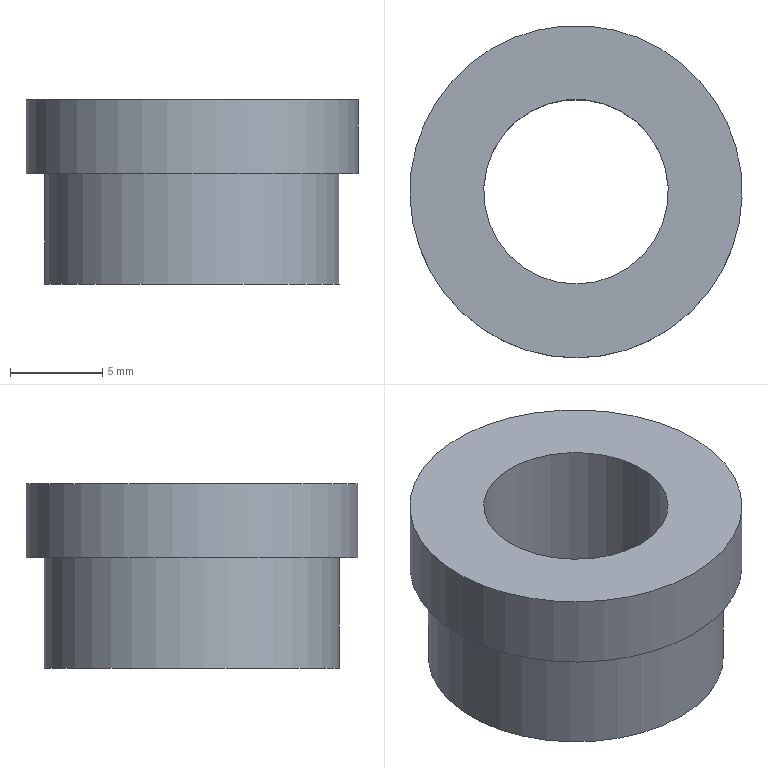Component | NX | GLAND | 1 solid | 6 faces | box 18 x 18 x 10 mm | volume 1341 mm3 | cylinder 3 | plane 2 | cone 1 | commonest cylinder face diameters 16 x1 10 x1 18 x1
STEP:
#1=CARTESIAN_POINT('',(0.,0.,0.));
#2=DIRECTION('',(0.,0.,1.));
#3=DIRECTION('',(1.,0.,0.));
#4=AXIS2_PLACEMENT_3D('',#1,#2,#3);
#5=CARTESIAN_POINT('',(10.284,-2.216,132.));
#6=VERTEX_POINT('',#5);
#7=CARTESIAN_POINT('',(10.284,5.784,132.));
#8=DIRECTION('',(0.,0.,1.));
#9=DIRECTION('',(0.,-1.,0.));
#10=AXIS2_PLACEMENT_3D('',#7,#8,#9);
#11=CIRCLE('',#10,8.);
#12=CARTESIAN_POINT('',(10.284,5.784,132.));
#13=DIRECTION('',(0.,0.,1.));
#14=DIRECTION('',(0.,-1.,0.));
#15=AXIS2_PLACEMENT_3D('',#12,#13,#14);
#16=CYLINDRICAL_SURFACE('',#15,8.);
#17=CARTESIAN_POINT('',(0.,0.));
#18=DIRECTION('',(1.,0.));
#19=VECTOR('',#18,1.);
#20=LINE('',#17,#19);
#21=(GEOMETRIC_REPRESENTATION_CONTEXT(2)PARAMETRIC_REPRESENTATION_CONTEXT()REPRESENTATION_CONTEXT('',''));
#22=DEFINITIONAL_REPRESENTATION('',(#20),#21);
#23=PCURVE('',#16,#22);
#24=CARTESIAN_POINT('',(10.284,5.784,132.));
#25=DIRECTION('',(0.,-0.,-1.));
#26=DIRECTION('',(0.,1.,-0.));
#27=AXIS2_PLACEMENT_3D('',#24,#25,#26);
#28=CONICAL_SURFACE('',#27,8.,1.047);
#29=CARTESIAN_POINT('',(9.425,0.));
#30=DIRECTION('',(-1.,0.));
#31=VECTOR('',#30,1.);
#32=LINE('',#29,#31);
#33=(GEOMETRIC_REPRESENTATION_CONTEXT(2)PARAMETRIC_REPRESENTATION_CONTEXT()REPRESENTATION_CONTEXT('',''));
#34=DEFINITIONAL_REPRESENTATION('',(#32),#33);
#35=PCURVE('',#28,#34);
#36=SURFACE_CURVE('',#11,(#23,#35),.PCURVE_S1.);
#37=EDGE_CURVE('',#6,#6,#36,.T.);
#38=ORIENTED_EDGE('',*,*,#37,.T.);
#39=CARTESIAN_POINT('',(10.284,-2.216,138.));
#40=VERTEX_POINT('',#39);
#41=CARTESIAN_POINT('',(10.284,-2.216,132.));
#42=CARTESIAN_POINT('',(10.284,-2.216,138.));
#43=B_SPLINE_CURVE_WITH_KNOTS('',1,(#41,#42),.UNSPECIFIED.,.F.,.F.,(2,2),(0.,6.),.PIECEWISE_BEZIER_KNOTS.);
#44=CARTESIAN_POINT('',(6.283,0.));
#45=DIRECTION('',(0.,1.));
#46=VECTOR('',#45,1.);
#47=LINE('',#44,#46);
#48=(GEOMETRIC_REPRESENTATION_CONTEXT(2)PARAMETRIC_REPRESENTATION_CONTEXT()REPRESENTATION_CONTEXT('',''));
#49=DEFINITIONAL_REPRESENTATION('',(#47),#48);
#50=PCURVE('',#16,#49);
#51=CARTESIAN_POINT('',(0.,0.));
#52=DIRECTION('',(0.,1.));
#53=VECTOR('',#52,1.);
#54=LINE('',#51,#53);
#55=(GEOMETRIC_REPRESENTATION_CONTEXT(2)PARAMETRIC_REPRESENTATION_CONTEXT()REPRESENTATION_CONTEXT('',''));
#56=DEFINITIONAL_REPRESENTATION('',(#54),#55);
#57=PCURVE('',#16,#56);
#58=SEAM_CURVE('',#43,(#50,#57),.PCURVE_S1.);
#59=EDGE_CURVE('',#6,#40,#58,.T.);
#60=ORIENTED_EDGE('',*,*,#59,.T.);
#61=CARTESIAN_POINT('',(10.284,5.784,138.));
#62=DIRECTION('',(0.,0.,1.));
#63=DIRECTION('',(0.,-1.,0.));
#64=AXIS2_PLACEMENT_3D('',#61,#62,#63);
#65=CIRCLE('',#64,8.);
#66=CARTESIAN_POINT('',(0.,6.));
#67=DIRECTION('',(1.,0.));
#68=VECTOR('',#67,1.);
#69=LINE('',#66,#68);
#70=(GEOMETRIC_REPRESENTATION_CONTEXT(2)PARAMETRIC_REPRESENTATION_CONTEXT()REPRESENTATION_CONTEXT('',''));
#71=DEFINITIONAL_REPRESENTATION('',(#69),#70);
#72=PCURVE('',#16,#71);
#73=CARTESIAN_POINT('',(10.284,14.784,138.));
#74=DIRECTION('',(0.,-0.,-1.));
#75=DIRECTION('',(0.,1.,-0.));
#76=AXIS2_PLACEMENT_3D('',#73,#74,#75);
#77=PLANE('',#76);
#78=CARTESIAN_POINT('',(-17.,0.));
#79=CARTESIAN_POINT('',(-17.,13.856));
#80=CARTESIAN_POINT('',(-5.,6.928));
#81=CARTESIAN_POINT('',(7.,0.));
#82=CARTESIAN_POINT('',(-5.,-6.928));
#83=CARTESIAN_POINT('',(-17.,-13.856));
#84=CARTESIAN_POINT('',(-17.,0.));
#85=(BOUNDED_CURVE()B_SPLINE_CURVE(2,(#78,#79,#80,#81,#82,#83,#84),.UNSPECIFIED.,.T.,.F.)B_SPLINE_CURVE_WITH_KNOTS((1,2,2,2,2,1),(-2.094,0.,2.094,4.189,6.283,8.378),.UNSPECIFIED.)CURVE()GEOMETRIC_REPRESENTATION_ITEM()RATIONAL_B_SPLINE_CURVE((1.,0.5,1.,0.5,1.,0.5,1.))REPRESENTATION_ITEM(''));
#86=(GEOMETRIC_REPRESENTATION_CONTEXT(2)PARAMETRIC_REPRESENTATION_CONTEXT()REPRESENTATION_CONTEXT('',''));
#87=DEFINITIONAL_REPRESENTATION('',(#85),#86);
#88=PCURVE('',#77,#87);
#89=SURFACE_CURVE('',#65,(#72,#88),.PCURVE_S1.);
#90=EDGE_CURVE('',#40,#40,#89,.T.);
#91=ORIENTED_EDGE('',*,*,#90,.F.);
#92=ORIENTED_EDGE('',*,*,#59,.F.);
#93=EDGE_LOOP('',(#38,#60,#91,#92));
#94=FACE_BOUND('',#93,.T.);
#95=ADVANCED_FACE('',(#94),#16,.T.);
#96=CARTESIAN_POINT('',(10.284,0.7843,133.732));
#97=VERTEX_POINT('',#96);
#98=CARTESIAN_POINT('',(10.284,5.784,133.732));
#99=DIRECTION('',(0.,0.,1.));
#100=DIRECTION('',(0.,-1.,0.));
#101=AXIS2_PLACEMENT_3D('',#98,#99,#100);
#102=CIRCLE('',#101,5.);
#103=CARTESIAN_POINT('',(9.425,-1.732));
#104=DIRECTION('',(-1.,0.));
#105=VECTOR('',#104,1.);
#106=LINE('',#103,#105);
#107=(GEOMETRIC_REPRESENTATION_CONTEXT(2)PARAMETRIC_REPRESENTATION_CONTEXT()REPRESENTATION_CONTEXT('',''));
#108=DEFINITIONAL_REPRESENTATION('',(#106),#107);
#109=PCURVE('',#28,#108);
#110=CARTESIAN_POINT('',(10.284,5.784,132.));
#111=DIRECTION('',(0.,0.,1.));
#112=DIRECTION('',(0.,-1.,0.));
#113=AXIS2_PLACEMENT_3D('',#110,#111,#112);
#114=CYLINDRICAL_SURFACE('',#113,5.);
#115=CARTESIAN_POINT('',(0.,1.732));
#116=DIRECTION('',(1.,0.));
#117=VECTOR('',#116,1.);
#118=LINE('',#115,#117);
#119=(GEOMETRIC_REPRESENTATION_CONTEXT(2)PARAMETRIC_REPRESENTATION_CONTEXT()REPRESENTATION_CONTEXT('',''));
#120=DEFINITIONAL_REPRESENTATION('',(#118),#119);
#121=PCURVE('',#114,#120);
#122=SURFACE_CURVE('',#102,(#109,#121),.PCURVE_S1.);
#123=EDGE_CURVE('',#97,#97,#122,.T.);
#124=ORIENTED_EDGE('',*,*,#123,.F.);
#125=CARTESIAN_POINT('',(10.284,0.7843,133.732));
#126=CARTESIAN_POINT('',(10.284,-2.216,132.));
#127=B_SPLINE_CURVE_WITH_KNOTS('',1,(#125,#126),.UNSPECIFIED.,.F.,.F.,(2,2),(-3.464,0.),.PIECEWISE_BEZIER_KNOTS.);
#128=CARTESIAN_POINT('',(9.425,0.));
#129=DIRECTION('',(0.,1.));
#130=VECTOR('',#129,1.);
#131=LINE('',#128,#130);
#132=(GEOMETRIC_REPRESENTATION_CONTEXT(2)PARAMETRIC_REPRESENTATION_CONTEXT()REPRESENTATION_CONTEXT('',''));
#133=DEFINITIONAL_REPRESENTATION('',(#131),#132);
#134=PCURVE('',#28,#133);
#135=CARTESIAN_POINT('',(3.142,0.));
#136=DIRECTION('',(0.,1.));
#137=VECTOR('',#136,1.);
#138=LINE('',#135,#137);
#139=(GEOMETRIC_REPRESENTATION_CONTEXT(2)PARAMETRIC_REPRESENTATION_CONTEXT()REPRESENTATION_CONTEXT('',''));
#140=DEFINITIONAL_REPRESENTATION('',(#138),#139);
#141=PCURVE('',#28,#140);
#142=SEAM_CURVE('',#127,(#134,#141),.PCURVE_S1.);
#143=EDGE_CURVE('',#97,#6,#142,.T.);
#144=ORIENTED_EDGE('',*,*,#143,.T.);
#145=ORIENTED_EDGE('',*,*,#37,.T.);
#146=ORIENTED_EDGE('',*,*,#143,.F.);
#147=EDGE_LOOP('',(#124,#144,#145,#146));
#148=FACE_BOUND('',#147,.F.);
#149=ADVANCED_FACE('',(#148),#28,.F.);
#150=CARTESIAN_POINT('',(10.284,0.7843,142.));
#151=VERTEX_POINT('',#150);
#152=CARTESIAN_POINT('',(10.284,5.784,142.));
#153=DIRECTION('',(0.,0.,1.));
#154=DIRECTION('',(0.,-1.,0.));
#155=AXIS2_PLACEMENT_3D('',#152,#153,#154);
#156=CIRCLE('',#155,5.);
#157=CARTESIAN_POINT('',(0.,10.));
#158=DIRECTION('',(1.,0.));
#159=VECTOR('',#158,1.);
#160=LINE('',#157,#159);
#161=(GEOMETRIC_REPRESENTATION_CONTEXT(2)PARAMETRIC_REPRESENTATION_CONTEXT()REPRESENTATION_CONTEXT('',''));
#162=DEFINITIONAL_REPRESENTATION('',(#160),#161);
#163=PCURVE('',#114,#162);
#164=CARTESIAN_POINT('',(10.284,10.784,142.));
#165=DIRECTION('',(0.,0.,1.));
#166=DIRECTION('',(0.,-1.,0.));
#167=AXIS2_PLACEMENT_3D('',#164,#165,#166);
#168=PLANE('',#167);
#169=CARTESIAN_POINT('',(5.,0.));
#170=DIRECTION('',(1.,0.));
#171=AXIS2_PLACEMENT_2D('',#169,#170);
#172=CIRCLE('',#171,5.);
#173=(GEOMETRIC_REPRESENTATION_CONTEXT(2)PARAMETRIC_REPRESENTATION_CONTEXT()REPRESENTATION_CONTEXT('',''));
#174=DEFINITIONAL_REPRESENTATION('',(#172),#173);
#175=PCURVE('',#168,#174);
#176=SURFACE_CURVE('',#156,(#163,#175),.PCURVE_S1.);
#177=EDGE_CURVE('',#151,#151,#176,.T.);
#178=ORIENTED_EDGE('',*,*,#177,.F.);
#179=CARTESIAN_POINT('',(10.284,0.7843,133.732));
#180=CARTESIAN_POINT('',(10.284,0.7843,142.));
#181=B_SPLINE_CURVE_WITH_KNOTS('',1,(#179,#180),.UNSPECIFIED.,.F.,.F.,(2,2),(1.732,10.),.PIECEWISE_BEZIER_KNOTS.);
#182=CARTESIAN_POINT('',(0.,0.));
#183=DIRECTION('',(0.,1.));
#184=VECTOR('',#183,1.);
#185=LINE('',#182,#184);
#186=(GEOMETRIC_REPRESENTATION_CONTEXT(2)PARAMETRIC_REPRESENTATION_CONTEXT()REPRESENTATION_CONTEXT('',''));
#187=DEFINITIONAL_REPRESENTATION('',(#185),#186);
#188=PCURVE('',#114,#187);
#189=CARTESIAN_POINT('',(6.283,0.));
#190=DIRECTION('',(0.,1.));
#191=VECTOR('',#190,1.);
#192=LINE('',#189,#191);
#193=(GEOMETRIC_REPRESENTATION_CONTEXT(2)PARAMETRIC_REPRESENTATION_CONTEXT()REPRESENTATION_CONTEXT('',''));
#194=DEFINITIONAL_REPRESENTATION('',(#192),#193);
#195=PCURVE('',#114,#194);
#196=SEAM_CURVE('',#181,(#188,#195),.PCURVE_S1.);
#197=EDGE_CURVE('',#97,#151,#196,.T.);
#198=ORIENTED_EDGE('',*,*,#197,.F.);
#199=ORIENTED_EDGE('',*,*,#123,.T.);
#200=ORIENTED_EDGE('',*,*,#197,.T.);
#201=EDGE_LOOP('',(#178,#198,#199,#200));
#202=FACE_BOUND('',#201,.F.);
#203=ADVANCED_FACE('',(#202),#114,.F.);
#204=CARTESIAN_POINT('',(10.284,-3.216,142.));
#205=VERTEX_POINT('',#204);
#206=CARTESIAN_POINT('',(10.284,5.784,142.));
#207=DIRECTION('',(0.,0.,1.));
#208=DIRECTION('',(0.,-1.,0.));
#209=AXIS2_PLACEMENT_3D('',#206,#207,#208);
#210=CIRCLE('',#209,9.);
#211=CARTESIAN_POINT('',(5.,0.));
#212=DIRECTION('',(1.,0.));
#213=AXIS2_PLACEMENT_2D('',#211,#212);
#214=CIRCLE('',#213,9.);
#215=(GEOMETRIC_REPRESENTATION_CONTEXT(2)PARAMETRIC_REPRESENTATION_CONTEXT()REPRESENTATION_CONTEXT('',''));
#216=DEFINITIONAL_REPRESENTATION('',(#214),#215);
#217=PCURVE('',#168,#216);
#218=CARTESIAN_POINT('',(10.284,5.784,132.));
#219=DIRECTION('',(0.,0.,1.));
#220=DIRECTION('',(0.,-1.,0.));
#221=AXIS2_PLACEMENT_3D('',#218,#219,#220);
#222=CYLINDRICAL_SURFACE('',#221,9.);
#223=CARTESIAN_POINT('',(0.,10.));
#224=DIRECTION('',(1.,0.));
#225=VECTOR('',#224,1.);
#226=LINE('',#223,#225);
#227=(GEOMETRIC_REPRESENTATION_CONTEXT(2)PARAMETRIC_REPRESENTATION_CONTEXT()REPRESENTATION_CONTEXT('',''));
#228=DEFINITIONAL_REPRESENTATION('',(#226),#227);
#229=PCURVE('',#222,#228);
#230=SURFACE_CURVE('',#210,(#217,#229),.PCURVE_S1.);
#231=EDGE_CURVE('',#205,#205,#230,.T.);
#232=ORIENTED_EDGE('',*,*,#231,.T.);
#233=EDGE_LOOP('',(#232));
#234=FACE_BOUND('',#233,.T.);
#235=ORIENTED_EDGE('',*,*,#177,.F.);
#236=EDGE_LOOP('',(#235));
#237=FACE_BOUND('',#236,.T.);
#238=ADVANCED_FACE('',(#234,#237),#168,.T.);
#239=CARTESIAN_POINT('',(10.284,-3.216,138.));
#240=VERTEX_POINT('',#239);
#241=CARTESIAN_POINT('',(10.284,5.784,138.));
#242=DIRECTION('',(0.,0.,1.));
#243=DIRECTION('',(0.,-1.,0.));
#244=AXIS2_PLACEMENT_3D('',#241,#242,#243);
#245=CIRCLE('',#244,9.);
#246=CARTESIAN_POINT('',(0.,6.));
#247=DIRECTION('',(1.,0.));
#248=VECTOR('',#247,1.);
#249=LINE('',#246,#248);
#250=(GEOMETRIC_REPRESENTATION_CONTEXT(2)PARAMETRIC_REPRESENTATION_CONTEXT()REPRESENTATION_CONTEXT('',''));
#251=DEFINITIONAL_REPRESENTATION('',(#249),#250);
#252=PCURVE('',#222,#251);
#253=CARTESIAN_POINT('',(-18.,0.));
#254=CARTESIAN_POINT('',(-18.,15.588));
#255=CARTESIAN_POINT('',(-4.5,7.794));
#256=CARTESIAN_POINT('',(9.,0.));
#257=CARTESIAN_POINT('',(-4.5,-7.794));
#258=CARTESIAN_POINT('',(-18.,-15.588));
#259=CARTESIAN_POINT('',(-18.,0.));
#260=(BOUNDED_CURVE()B_SPLINE_CURVE(2,(#253,#254,#255,#256,#257,#258,#259),.UNSPECIFIED.,.T.,.F.)B_SPLINE_CURVE_WITH_KNOTS((1,2,2,2,2,1),(-2.094,0.,2.094,4.189,6.283,8.378),.UNSPECIFIED.)CURVE()GEOMETRIC_REPRESENTATION_ITEM()RATIONAL_B_SPLINE_CURVE((1.,0.5,1.,0.5,1.,0.5,1.))REPRESENTATION_ITEM(''));
#261=(GEOMETRIC_REPRESENTATION_CONTEXT(2)PARAMETRIC_REPRESENTATION_CONTEXT()REPRESENTATION_CONTEXT('',''));
#262=DEFINITIONAL_REPRESENTATION('',(#260),#261);
#263=PCURVE('',#77,#262);
#264=SURFACE_CURVE('',#245,(#252,#263),.PCURVE_S1.);
#265=EDGE_CURVE('',#240,#240,#264,.T.);
#266=ORIENTED_EDGE('',*,*,#265,.T.);
#267=CARTESIAN_POINT('',(10.284,-3.216,138.));
#268=CARTESIAN_POINT('',(10.284,-3.216,142.));
#269=B_SPLINE_CURVE_WITH_KNOTS('',1,(#267,#268),.UNSPECIFIED.,.F.,.F.,(2,2),(6.,10.),.PIECEWISE_BEZIER_KNOTS.);
#270=CARTESIAN_POINT('',(6.283,0.));
#271=DIRECTION('',(0.,1.));
#272=VECTOR('',#271,1.);
#273=LINE('',#270,#272);
#274=(GEOMETRIC_REPRESENTATION_CONTEXT(2)PARAMETRIC_REPRESENTATION_CONTEXT()REPRESENTATION_CONTEXT('',''));
#275=DEFINITIONAL_REPRESENTATION('',(#273),#274);
#276=PCURVE('',#222,#275);
#277=CARTESIAN_POINT('',(0.,0.));
#278=DIRECTION('',(0.,1.));
#279=VECTOR('',#278,1.);
#280=LINE('',#277,#279);
#281=(GEOMETRIC_REPRESENTATION_CONTEXT(2)PARAMETRIC_REPRESENTATION_CONTEXT()REPRESENTATION_CONTEXT('',''));
#282=DEFINITIONAL_REPRESENTATION('',(#280),#281);
#283=PCURVE('',#222,#282);
#284=SEAM_CURVE('',#269,(#276,#283),.PCURVE_S1.);
#285=EDGE_CURVE('',#240,#205,#284,.T.);
#286=ORIENTED_EDGE('',*,*,#285,.T.);
#287=ORIENTED_EDGE('',*,*,#231,.F.);
#288=ORIENTED_EDGE('',*,*,#285,.F.);
#289=EDGE_LOOP('',(#266,#286,#287,#288));
#290=FACE_BOUND('',#289,.T.);
#291=ADVANCED_FACE('',(#290),#222,.T.);
#292=ORIENTED_EDGE('',*,*,#90,.T.);
#293=EDGE_LOOP('',(#292));
#294=FACE_BOUND('',#293,.T.);
#295=ORIENTED_EDGE('',*,*,#265,.F.);
#296=EDGE_LOOP('',(#295));
#297=FACE_BOUND('',#296,.T.);
#298=ADVANCED_FACE('',(#294,#297),#77,.T.);
#299=CLOSED_SHELL('',(#95,#149,#203,#238,#291,#298));
#300=MANIFOLD_SOLID_BREP('',#299);
#301=(LENGTH_UNIT()NAMED_UNIT(*)SI_UNIT(.MILLI.,.METRE.));
#302=UNCERTAINTY_MEASURE_WITH_UNIT(LENGTH_MEASURE(0.00001),#301,'','');
#303=(NAMED_UNIT(*)PLANE_ANGLE_UNIT()SI_UNIT($,.RADIAN.));
#304=(NAMED_UNIT(*)SI_UNIT($,.STERADIAN.)SOLID_ANGLE_UNIT());
#305=(GEOMETRIC_REPRESENTATION_CONTEXT(3)GLOBAL_UNCERTAINTY_ASSIGNED_CONTEXT((#302))GLOBAL_UNIT_ASSIGNED_CONTEXT((#301,#303,#304))REPRESENTATION_CONTEXT('',''));
#306=ADVANCED_BREP_SHAPE_REPRESENTATION('',(#4,#300),#305);